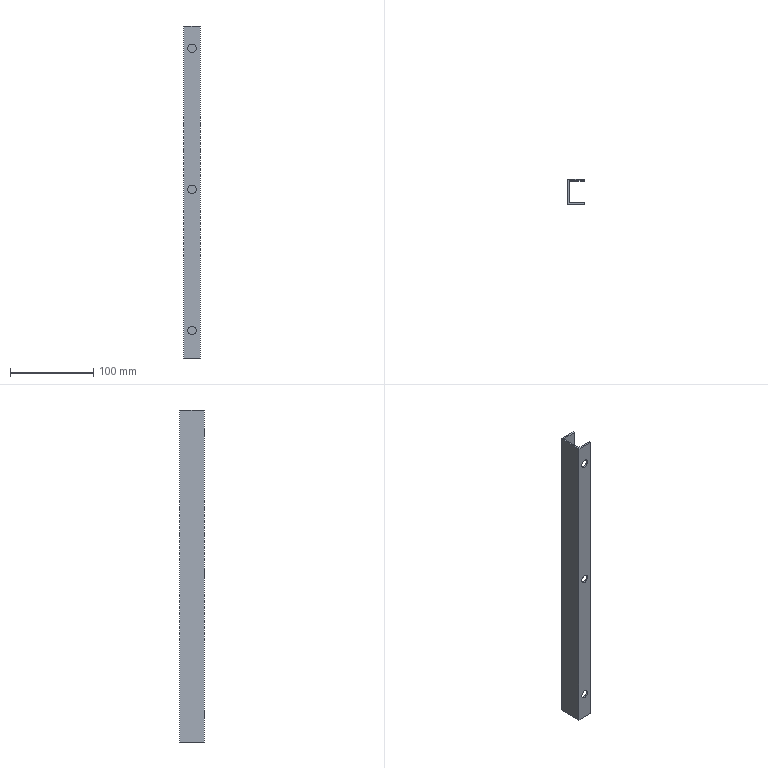Component | SolidWorks | Mirror Part3^Assembly2-4 | 1 solid | 16 faces | box 20 x 30 x 400 mm | volume 52329 mm3 | plane 10 | cylinder 6 | commonest cylinder face diameters 10 x6
STEP:
#1=CARTESIAN_POINT('',(-5.787,0.07874,-30.249));
#2=VERTEX_POINT('',#1);
#3=CARTESIAN_POINT('',(-5.394,0.07874,-30.249));
#4=VERTEX_POINT('',#3);
#5=CARTESIAN_POINT('',(-5.591,0.07874,-30.249));
#6=DIRECTION('',(0.,1.,0.));
#7=DIRECTION('',(-1.,0.,0.));
#8=AXIS2_PLACEMENT_3D('',#5,#6,#7);
#9=CIRCLE('',#8,0.1969);
#10=EDGE_CURVE('',#2,#4,#9,.T.);
#11=ORIENTED_EDGE('',*,*,#10,.T.);
#12=CARTESIAN_POINT('',(-5.394,0.,-30.249));
#13=VERTEX_POINT('',#12);
#14=CARTESIAN_POINT('',(-5.394,0.1969,-30.249));
#15=DIRECTION('',(-0.,-1.,0.));
#16=VECTOR('',#15,39.37);
#17=LINE('',#14,#16);
#18=EDGE_CURVE('',#4,#13,#17,.T.);
#19=ORIENTED_EDGE('',*,*,#18,.T.);
#20=CARTESIAN_POINT('',(-5.787,0.,-30.249));
#21=VERTEX_POINT('',#20);
#22=CARTESIAN_POINT('',(-5.591,0.,-30.249));
#23=DIRECTION('',(0.,1.,0.));
#24=DIRECTION('',(-1.,0.,0.));
#25=AXIS2_PLACEMENT_3D('',#22,#23,#24);
#26=CIRCLE('',#25,0.1969);
#27=EDGE_CURVE('',#21,#13,#26,.T.);
#28=ORIENTED_EDGE('',*,*,#27,.F.);
#29=CARTESIAN_POINT('',(-5.787,0.1969,-30.249));
#30=DIRECTION('',(-0.,-1.,0.));
#31=VECTOR('',#30,39.37);
#32=LINE('',#29,#31);
#33=EDGE_CURVE('',#2,#21,#32,.T.);
#34=ORIENTED_EDGE('',*,*,#33,.F.);
#35=EDGE_LOOP('',(#11,#19,#28,#34));
#36=FACE_OUTER_BOUND('',#35,.T.);
#37=CARTESIAN_POINT('',(-5.591,0.1969,-30.249));
#38=DIRECTION('',(-0.,-1.,0.));
#39=DIRECTION('',(-1.,0.,0.));
#40=AXIS2_PLACEMENT_3D('',#37,#38,#39);
#41=CYLINDRICAL_SURFACE('',#40,0.1969);
#42=ADVANCED_FACE('',(#36),#41,.F.);
#43=CARTESIAN_POINT('',(-5.787,0.07874,-23.556));
#44=VERTEX_POINT('',#43);
#45=CARTESIAN_POINT('',(-5.394,0.07874,-23.556));
#46=VERTEX_POINT('',#45);
#47=CARTESIAN_POINT('',(-5.591,0.07874,-23.556));
#48=DIRECTION('',(0.,1.,0.));
#49=DIRECTION('',(-1.,0.,0.));
#50=AXIS2_PLACEMENT_3D('',#47,#48,#49);
#51=CIRCLE('',#50,0.1969);
#52=EDGE_CURVE('',#44,#46,#51,.T.);
#53=ORIENTED_EDGE('',*,*,#52,.T.);
#54=CARTESIAN_POINT('',(-5.394,0.,-23.556));
#55=VERTEX_POINT('',#54);
#56=CARTESIAN_POINT('',(-5.394,0.1969,-23.556));
#57=DIRECTION('',(-0.,-1.,0.));
#58=VECTOR('',#57,39.37);
#59=LINE('',#56,#58);
#60=EDGE_CURVE('',#46,#55,#59,.T.);
#61=ORIENTED_EDGE('',*,*,#60,.T.);
#62=CARTESIAN_POINT('',(-5.787,0.,-23.556));
#63=VERTEX_POINT('',#62);
#64=CARTESIAN_POINT('',(-5.591,0.,-23.556));
#65=DIRECTION('',(0.,1.,0.));
#66=DIRECTION('',(-1.,0.,0.));
#67=AXIS2_PLACEMENT_3D('',#64,#65,#66);
#68=CIRCLE('',#67,0.1969);
#69=EDGE_CURVE('',#63,#55,#68,.T.);
#70=ORIENTED_EDGE('',*,*,#69,.F.);
#71=CARTESIAN_POINT('',(-5.787,0.1969,-23.556));
#72=DIRECTION('',(-0.,-1.,0.));
#73=VECTOR('',#72,39.37);
#74=LINE('',#71,#73);
#75=EDGE_CURVE('',#44,#63,#74,.T.);
#76=ORIENTED_EDGE('',*,*,#75,.F.);
#77=EDGE_LOOP('',(#53,#61,#70,#76));
#78=FACE_OUTER_BOUND('',#77,.T.);
#79=CARTESIAN_POINT('',(-5.591,0.1969,-23.556));
#80=DIRECTION('',(-0.,-1.,0.));
#81=DIRECTION('',(-1.,0.,0.));
#82=AXIS2_PLACEMENT_3D('',#79,#80,#81);
#83=CYLINDRICAL_SURFACE('',#82,0.1969);
#84=ADVANCED_FACE('',(#78),#83,.F.);
#85=CARTESIAN_POINT('',(-5.787,0.07874,-16.863));
#86=VERTEX_POINT('',#85);
#87=CARTESIAN_POINT('',(-5.394,0.07874,-16.863));
#88=VERTEX_POINT('',#87);
#89=CARTESIAN_POINT('',(-5.591,0.07874,-16.863));
#90=DIRECTION('',(0.,1.,0.));
#91=DIRECTION('',(-1.,0.,0.));
#92=AXIS2_PLACEMENT_3D('',#89,#90,#91);
#93=CIRCLE('',#92,0.1969);
#94=EDGE_CURVE('',#86,#88,#93,.T.);
#95=ORIENTED_EDGE('',*,*,#94,.T.);
#96=CARTESIAN_POINT('',(-5.394,0.,-16.863));
#97=VERTEX_POINT('',#96);
#98=CARTESIAN_POINT('',(-5.394,0.1969,-16.863));
#99=DIRECTION('',(-0.,-1.,0.));
#100=VECTOR('',#99,39.37);
#101=LINE('',#98,#100);
#102=EDGE_CURVE('',#88,#97,#101,.T.);
#103=ORIENTED_EDGE('',*,*,#102,.T.);
#104=CARTESIAN_POINT('',(-5.787,0.,-16.863));
#105=VERTEX_POINT('',#104);
#106=CARTESIAN_POINT('',(-5.591,0.,-16.863));
#107=DIRECTION('',(0.,1.,0.));
#108=DIRECTION('',(-1.,0.,0.));
#109=AXIS2_PLACEMENT_3D('',#106,#107,#108);
#110=CIRCLE('',#109,0.1969);
#111=EDGE_CURVE('',#105,#97,#110,.T.);
#112=ORIENTED_EDGE('',*,*,#111,.F.);
#113=CARTESIAN_POINT('',(-5.787,0.1969,-16.863));
#114=DIRECTION('',(-0.,-1.,0.));
#115=VECTOR('',#114,39.37);
#116=LINE('',#113,#115);
#117=EDGE_CURVE('',#86,#105,#116,.T.);
#118=ORIENTED_EDGE('',*,*,#117,.F.);
#119=EDGE_LOOP('',(#95,#103,#112,#118));
#120=FACE_OUTER_BOUND('',#119,.T.);
#121=CARTESIAN_POINT('',(-5.591,0.1969,-16.863));
#122=DIRECTION('',(-0.,-1.,0.));
#123=DIRECTION('',(-1.,0.,0.));
#124=AXIS2_PLACEMENT_3D('',#121,#122,#123);
#125=CYLINDRICAL_SURFACE('',#124,0.1969);
#126=ADVANCED_FACE('',(#120),#125,.F.);
#127=ORIENTED_EDGE('',*,*,#10,.F.);
#128=CARTESIAN_POINT('',(-5.591,0.07874,-30.249));
#129=DIRECTION('',(0.,1.,0.));
#130=DIRECTION('',(-1.,0.,0.));
#131=AXIS2_PLACEMENT_3D('',#128,#129,#130);
#132=CIRCLE('',#131,0.1969);
#133=EDGE_CURVE('',#4,#2,#132,.T.);
#134=ORIENTED_EDGE('',*,*,#133,.F.);
#135=EDGE_LOOP('',(#127,#134));
#136=FACE_BOUND('',#135,.T.);
#137=ORIENTED_EDGE('',*,*,#52,.F.);
#138=CARTESIAN_POINT('',(-5.591,0.07874,-23.556));
#139=DIRECTION('',(0.,1.,0.));
#140=DIRECTION('',(-1.,0.,0.));
#141=AXIS2_PLACEMENT_3D('',#138,#139,#140);
#142=CIRCLE('',#141,0.1969);
#143=EDGE_CURVE('',#46,#44,#142,.T.);
#144=ORIENTED_EDGE('',*,*,#143,.F.);
#145=EDGE_LOOP('',(#137,#144));
#146=FACE_BOUND('',#145,.T.);
#147=ORIENTED_EDGE('',*,*,#94,.F.);
#148=CARTESIAN_POINT('',(-5.591,0.07874,-16.863));
#149=DIRECTION('',(0.,1.,0.));
#150=DIRECTION('',(-1.,0.,0.));
#151=AXIS2_PLACEMENT_3D('',#148,#149,#150);
#152=CIRCLE('',#151,0.1969);
#153=EDGE_CURVE('',#88,#86,#152,.T.);
#154=ORIENTED_EDGE('',*,*,#153,.F.);
#155=EDGE_LOOP('',(#147,#154));
#156=FACE_BOUND('',#155,.T.);
#157=CARTESIAN_POINT('',(-5.906,0.07874,-31.557));
#158=VERTEX_POINT('',#157);
#159=CARTESIAN_POINT('',(-5.197,0.07874,-31.557));
#160=VERTEX_POINT('',#159);
#161=CARTESIAN_POINT('',(-5.984,0.07874,-31.557));
#162=DIRECTION('',(1.,-0.,0.));
#163=VECTOR('',#162,39.37);
#164=LINE('',#161,#163);
#165=EDGE_CURVE('',#158,#160,#164,.T.);
#166=ORIENTED_EDGE('',*,*,#165,.F.);
#167=CARTESIAN_POINT('',(-5.906,0.07874,-15.809));
#168=VERTEX_POINT('',#167);
#169=CARTESIAN_POINT('',(-5.906,0.07874,-15.809));
#170=DIRECTION('',(0.,0.,-1.));
#171=VECTOR('',#170,39.37);
#172=LINE('',#169,#171);
#173=EDGE_CURVE('',#168,#158,#172,.T.);
#174=ORIENTED_EDGE('',*,*,#173,.F.);
#175=CARTESIAN_POINT('',(-5.197,0.07874,-15.809));
#176=VERTEX_POINT('',#175);
#177=CARTESIAN_POINT('',(-5.984,0.07874,-15.809));
#178=DIRECTION('',(1.,-0.,0.));
#179=VECTOR('',#178,39.37);
#180=LINE('',#177,#179);
#181=EDGE_CURVE('',#168,#176,#180,.T.);
#182=ORIENTED_EDGE('',*,*,#181,.T.);
#183=CARTESIAN_POINT('',(-5.197,0.07874,-15.809));
#184=DIRECTION('',(0.,0.,-1.));
#185=VECTOR('',#184,39.37);
#186=LINE('',#183,#185);
#187=EDGE_CURVE('',#176,#160,#186,.T.);
#188=ORIENTED_EDGE('',*,*,#187,.T.);
#189=EDGE_LOOP('',(#166,#174,#182,#188));
#190=FACE_OUTER_BOUND('',#189,.T.);
#191=CARTESIAN_POINT('',(-5.984,0.07874,-15.809));
#192=DIRECTION('',(-0.,-1.,0.));
#193=DIRECTION('',(-1.,0.,0.));
#194=AXIS2_PLACEMENT_3D('',#191,#192,#193);
#195=PLANE('',#194);
#196=ADVANCED_FACE('',(#136,#146,#156,#190),#195,.F.);
#197=CARTESIAN_POINT('',(-5.197,0.,-31.557));
#198=VERTEX_POINT('',#197);
#199=CARTESIAN_POINT('',(-5.197,0.,-31.557));
#200=DIRECTION('',(0.,1.,0.));
#201=VECTOR('',#200,39.37);
#202=LINE('',#199,#201);
#203=EDGE_CURVE('',#198,#160,#202,.T.);
#204=ORIENTED_EDGE('',*,*,#203,.T.);
#205=ORIENTED_EDGE('',*,*,#187,.F.);
#206=CARTESIAN_POINT('',(-5.197,0.,-15.809));
#207=VERTEX_POINT('',#206);
#208=CARTESIAN_POINT('',(-5.197,0.,-15.809));
#209=DIRECTION('',(0.,1.,0.));
#210=VECTOR('',#209,39.37);
#211=LINE('',#208,#210);
#212=EDGE_CURVE('',#207,#176,#211,.T.);
#213=ORIENTED_EDGE('',*,*,#212,.F.);
#214=CARTESIAN_POINT('',(-5.197,0.,-15.809));
#215=DIRECTION('',(0.,0.,-1.));
#216=VECTOR('',#215,39.37);
#217=LINE('',#214,#216);
#218=EDGE_CURVE('',#207,#198,#217,.T.);
#219=ORIENTED_EDGE('',*,*,#218,.T.);
#220=EDGE_LOOP('',(#204,#205,#213,#219));
#221=FACE_OUTER_BOUND('',#220,.T.);
#222=CARTESIAN_POINT('',(-5.197,0.,-15.809));
#223=DIRECTION('',(1.,0.,0.));
#224=DIRECTION('',(0.,0.,1.));
#225=AXIS2_PLACEMENT_3D('',#222,#223,#224);
#226=PLANE('',#225);
#227=ADVANCED_FACE('',(#221),#226,.T.);
#228=ORIENTED_EDGE('',*,*,#27,.T.);
#229=CARTESIAN_POINT('',(-5.591,0.,-30.249));
#230=DIRECTION('',(0.,1.,0.));
#231=DIRECTION('',(-1.,0.,0.));
#232=AXIS2_PLACEMENT_3D('',#229,#230,#231);
#233=CIRCLE('',#232,0.1969);
#234=EDGE_CURVE('',#13,#21,#233,.T.);
#235=ORIENTED_EDGE('',*,*,#234,.T.);
#236=EDGE_LOOP('',(#228,#235));
#237=FACE_BOUND('',#236,.T.);
#238=ORIENTED_EDGE('',*,*,#69,.T.);
#239=CARTESIAN_POINT('',(-5.591,0.,-23.556));
#240=DIRECTION('',(0.,1.,0.));
#241=DIRECTION('',(-1.,0.,0.));
#242=AXIS2_PLACEMENT_3D('',#239,#240,#241);
#243=CIRCLE('',#242,0.1969);
#244=EDGE_CURVE('',#55,#63,#243,.T.);
#245=ORIENTED_EDGE('',*,*,#244,.T.);
#246=EDGE_LOOP('',(#238,#245));
#247=FACE_BOUND('',#246,.T.);
#248=ORIENTED_EDGE('',*,*,#111,.T.);
#249=CARTESIAN_POINT('',(-5.591,0.,-16.863));
#250=DIRECTION('',(0.,1.,0.));
#251=DIRECTION('',(-1.,0.,0.));
#252=AXIS2_PLACEMENT_3D('',#249,#250,#251);
#253=CIRCLE('',#252,0.1969);
#254=EDGE_CURVE('',#97,#105,#253,.T.);
#255=ORIENTED_EDGE('',*,*,#254,.T.);
#256=EDGE_LOOP('',(#248,#255));
#257=FACE_BOUND('',#256,.T.);
#258=CARTESIAN_POINT('',(-5.984,0.,-31.557));
#259=VERTEX_POINT('',#258);
#260=CARTESIAN_POINT('',(-5.984,0.,-31.557));
#261=DIRECTION('',(1.,-0.,0.));
#262=VECTOR('',#261,39.37);
#263=LINE('',#260,#262);
#264=EDGE_CURVE('',#259,#198,#263,.T.);
#265=ORIENTED_EDGE('',*,*,#264,.T.);
#266=ORIENTED_EDGE('',*,*,#218,.F.);
#267=CARTESIAN_POINT('',(-5.984,0.,-15.809));
#268=VERTEX_POINT('',#267);
#269=CARTESIAN_POINT('',(-5.984,0.,-15.809));
#270=DIRECTION('',(1.,-0.,0.));
#271=VECTOR('',#270,39.37);
#272=LINE('',#269,#271);
#273=EDGE_CURVE('',#268,#207,#272,.T.);
#274=ORIENTED_EDGE('',*,*,#273,.F.);
#275=CARTESIAN_POINT('',(-5.984,0.,-15.809));
#276=DIRECTION('',(0.,0.,-1.));
#277=VECTOR('',#276,39.37);
#278=LINE('',#275,#277);
#279=EDGE_CURVE('',#268,#259,#278,.T.);
#280=ORIENTED_EDGE('',*,*,#279,.T.);
#281=EDGE_LOOP('',(#265,#266,#274,#280));
#282=FACE_OUTER_BOUND('',#281,.T.);
#283=CARTESIAN_POINT('',(-5.984,0.,-15.809));
#284=DIRECTION('',(-0.,-1.,0.));
#285=DIRECTION('',(-1.,0.,0.));
#286=AXIS2_PLACEMENT_3D('',#283,#284,#285);
#287=PLANE('',#286);
#288=ADVANCED_FACE('',(#237,#247,#257,#282),#287,.T.);
#289=CARTESIAN_POINT('',(-5.984,1.181,-31.557));
#290=VERTEX_POINT('',#289);
#291=CARTESIAN_POINT('',(-5.984,0.,-31.557));
#292=DIRECTION('',(0.,-1.,0.));
#293=VECTOR('',#292,39.37);
#294=LINE('',#291,#293);
#295=EDGE_CURVE('',#290,#259,#294,.T.);
#296=ORIENTED_EDGE('',*,*,#295,.T.);
#297=ORIENTED_EDGE('',*,*,#279,.F.);
#298=CARTESIAN_POINT('',(-5.984,1.181,-15.809));
#299=VERTEX_POINT('',#298);
#300=CARTESIAN_POINT('',(-5.984,0.,-15.809));
#301=DIRECTION('',(0.,-1.,0.));
#302=VECTOR('',#301,39.37);
#303=LINE('',#300,#302);
#304=EDGE_CURVE('',#299,#268,#303,.T.);
#305=ORIENTED_EDGE('',*,*,#304,.F.);
#306=CARTESIAN_POINT('',(-5.984,1.181,-15.809));
#307=DIRECTION('',(0.,0.,-1.));
#308=VECTOR('',#307,39.37);
#309=LINE('',#306,#308);
#310=EDGE_CURVE('',#299,#290,#309,.T.);
#311=ORIENTED_EDGE('',*,*,#310,.T.);
#312=EDGE_LOOP('',(#296,#297,#305,#311));
#313=FACE_OUTER_BOUND('',#312,.T.);
#314=CARTESIAN_POINT('',(-5.984,0.,-15.809));
#315=DIRECTION('',(-1.,0.,0.));
#316=DIRECTION('',(0.,0.,-1.));
#317=AXIS2_PLACEMENT_3D('',#314,#315,#316);
#318=PLANE('',#317);
#319=ADVANCED_FACE('',(#313),#318,.T.);
#320=CARTESIAN_POINT('',(-5.197,1.181,-31.557));
#321=VERTEX_POINT('',#320);
#322=CARTESIAN_POINT('',(-5.984,1.181,-31.557));
#323=DIRECTION('',(-1.,0.,0.));
#324=VECTOR('',#323,39.37);
#325=LINE('',#322,#324);
#326=EDGE_CURVE('',#321,#290,#325,.T.);
#327=ORIENTED_EDGE('',*,*,#326,.T.);
#328=ORIENTED_EDGE('',*,*,#310,.F.);
#329=CARTESIAN_POINT('',(-5.197,1.181,-15.809));
#330=VERTEX_POINT('',#329);
#331=CARTESIAN_POINT('',(-5.984,1.181,-15.809));
#332=DIRECTION('',(-1.,0.,0.));
#333=VECTOR('',#332,39.37);
#334=LINE('',#331,#333);
#335=EDGE_CURVE('',#330,#299,#334,.T.);
#336=ORIENTED_EDGE('',*,*,#335,.F.);
#337=CARTESIAN_POINT('',(-5.197,1.181,-15.809));
#338=DIRECTION('',(0.,0.,-1.));
#339=VECTOR('',#338,39.37);
#340=LINE('',#337,#339);
#341=EDGE_CURVE('',#330,#321,#340,.T.);
#342=ORIENTED_EDGE('',*,*,#341,.T.);
#343=EDGE_LOOP('',(#327,#328,#336,#342));
#344=FACE_OUTER_BOUND('',#343,.T.);
#345=CARTESIAN_POINT('',(-5.984,1.181,-15.809));
#346=DIRECTION('',(0.,1.,0.));
#347=DIRECTION('',(0.,0.,1.));
#348=AXIS2_PLACEMENT_3D('',#345,#346,#347);
#349=PLANE('',#348);
#350=ADVANCED_FACE('',(#344),#349,.T.);
#351=CARTESIAN_POINT('',(-5.197,1.102,-31.557));
#352=VERTEX_POINT('',#351);
#353=CARTESIAN_POINT('',(-5.197,1.102,-31.557));
#354=DIRECTION('',(0.,1.,0.));
#355=VECTOR('',#354,39.37);
#356=LINE('',#353,#355);
#357=EDGE_CURVE('',#352,#321,#356,.T.);
#358=ORIENTED_EDGE('',*,*,#357,.T.);
#359=ORIENTED_EDGE('',*,*,#341,.F.);
#360=CARTESIAN_POINT('',(-5.197,1.102,-15.809));
#361=VERTEX_POINT('',#360);
#362=CARTESIAN_POINT('',(-5.197,1.102,-15.809));
#363=DIRECTION('',(0.,1.,0.));
#364=VECTOR('',#363,39.37);
#365=LINE('',#362,#364);
#366=EDGE_CURVE('',#361,#330,#365,.T.);
#367=ORIENTED_EDGE('',*,*,#366,.F.);
#368=CARTESIAN_POINT('',(-5.197,1.102,-15.809));
#369=DIRECTION('',(0.,0.,-1.));
#370=VECTOR('',#369,39.37);
#371=LINE('',#368,#370);
#372=EDGE_CURVE('',#361,#352,#371,.T.);
#373=ORIENTED_EDGE('',*,*,#372,.T.);
#374=EDGE_LOOP('',(#358,#359,#367,#373));
#375=FACE_OUTER_BOUND('',#374,.T.);
#376=CARTESIAN_POINT('',(-5.197,1.102,-15.809));
#377=DIRECTION('',(1.,0.,0.));
#378=DIRECTION('',(0.,0.,1.));
#379=AXIS2_PLACEMENT_3D('',#376,#377,#378);
#380=PLANE('',#379);
#381=ADVANCED_FACE('',(#375),#380,.T.);
#382=CARTESIAN_POINT('',(-5.906,1.102,-31.557));
#383=VERTEX_POINT('',#382);
#384=CARTESIAN_POINT('',(-5.984,1.102,-31.557));
#385=DIRECTION('',(-1.,0.,0.));
#386=VECTOR('',#385,39.37);
#387=LINE('',#384,#386);
#388=EDGE_CURVE('',#352,#383,#387,.T.);
#389=ORIENTED_EDGE('',*,*,#388,.F.);
#390=ORIENTED_EDGE('',*,*,#372,.F.);
#391=CARTESIAN_POINT('',(-5.906,1.102,-15.809));
#392=VERTEX_POINT('',#391);
#393=CARTESIAN_POINT('',(-5.984,1.102,-15.809));
#394=DIRECTION('',(-1.,0.,0.));
#395=VECTOR('',#394,39.37);
#396=LINE('',#393,#395);
#397=EDGE_CURVE('',#361,#392,#396,.T.);
#398=ORIENTED_EDGE('',*,*,#397,.T.);
#399=CARTESIAN_POINT('',(-5.906,1.102,-15.809));
#400=DIRECTION('',(0.,0.,-1.));
#401=VECTOR('',#400,39.37);
#402=LINE('',#399,#401);
#403=EDGE_CURVE('',#392,#383,#402,.T.);
#404=ORIENTED_EDGE('',*,*,#403,.T.);
#405=EDGE_LOOP('',(#389,#390,#398,#404));
#406=FACE_OUTER_BOUND('',#405,.T.);
#407=CARTESIAN_POINT('',(-5.984,1.102,-15.809));
#408=DIRECTION('',(0.,1.,0.));
#409=DIRECTION('',(0.,0.,1.));
#410=AXIS2_PLACEMENT_3D('',#407,#408,#409);
#411=PLANE('',#410);
#412=ADVANCED_FACE('',(#406),#411,.F.);
#413=CARTESIAN_POINT('',(-5.906,0.,-31.557));
#414=DIRECTION('',(0.,-1.,0.));
#415=VECTOR('',#414,39.37);
#416=LINE('',#413,#415);
#417=EDGE_CURVE('',#383,#158,#416,.T.);
#418=ORIENTED_EDGE('',*,*,#417,.F.);
#419=ORIENTED_EDGE('',*,*,#403,.F.);
#420=CARTESIAN_POINT('',(-5.906,0.,-15.809));
#421=DIRECTION('',(0.,-1.,0.));
#422=VECTOR('',#421,39.37);
#423=LINE('',#420,#422);
#424=EDGE_CURVE('',#392,#168,#423,.T.);
#425=ORIENTED_EDGE('',*,*,#424,.T.);
#426=ORIENTED_EDGE('',*,*,#173,.T.);
#427=EDGE_LOOP('',(#418,#419,#425,#426));
#428=FACE_OUTER_BOUND('',#427,.T.);
#429=CARTESIAN_POINT('',(-5.906,0.,-15.809));
#430=DIRECTION('',(-1.,0.,0.));
#431=DIRECTION('',(0.,0.,-1.));
#432=AXIS2_PLACEMENT_3D('',#429,#430,#431);
#433=PLANE('',#432);
#434=ADVANCED_FACE('',(#428),#433,.F.);
#435=ORIENTED_EDGE('',*,*,#181,.F.);
#436=ORIENTED_EDGE('',*,*,#424,.F.);
#437=ORIENTED_EDGE('',*,*,#397,.F.);
#438=ORIENTED_EDGE('',*,*,#366,.T.);
#439=ORIENTED_EDGE('',*,*,#335,.T.);
#440=ORIENTED_EDGE('',*,*,#304,.T.);
#441=ORIENTED_EDGE('',*,*,#273,.T.);
#442=ORIENTED_EDGE('',*,*,#212,.T.);
#443=EDGE_LOOP('',(#435,#436,#437,#438,#439,#440,#441,#442));
#444=FACE_OUTER_BOUND('',#443,.T.);
#445=CARTESIAN_POINT('',(-5.984,0.5561,-15.809));
#446=DIRECTION('',(0.,0.,-1.));
#447=DIRECTION('',(1.,0.,0.));
#448=AXIS2_PLACEMENT_3D('',#445,#446,#447);
#449=PLANE('',#448);
#450=ADVANCED_FACE('',(#444),#449,.F.);
#451=ORIENTED_EDGE('',*,*,#165,.T.);
#452=ORIENTED_EDGE('',*,*,#203,.F.);
#453=ORIENTED_EDGE('',*,*,#264,.F.);
#454=ORIENTED_EDGE('',*,*,#295,.F.);
#455=ORIENTED_EDGE('',*,*,#326,.F.);
#456=ORIENTED_EDGE('',*,*,#357,.F.);
#457=ORIENTED_EDGE('',*,*,#388,.T.);
#458=ORIENTED_EDGE('',*,*,#417,.T.);
#459=EDGE_LOOP('',(#451,#452,#453,#454,#455,#456,#457,#458));
#460=FACE_OUTER_BOUND('',#459,.T.);
#461=CARTESIAN_POINT('',(-5.984,0.5561,-31.557));
#462=DIRECTION('',(0.,0.,-1.));
#463=DIRECTION('',(1.,0.,0.));
#464=AXIS2_PLACEMENT_3D('',#461,#462,#463);
#465=PLANE('',#464);
#466=ADVANCED_FACE('',(#460),#465,.T.);
#467=ORIENTED_EDGE('',*,*,#102,.F.);
#468=ORIENTED_EDGE('',*,*,#153,.T.);
#469=ORIENTED_EDGE('',*,*,#117,.T.);
#470=ORIENTED_EDGE('',*,*,#254,.F.);
#471=EDGE_LOOP('',(#467,#468,#469,#470));
#472=FACE_OUTER_BOUND('',#471,.T.);
#473=CARTESIAN_POINT('',(-5.591,0.1969,-16.863));
#474=DIRECTION('',(-0.,-1.,0.));
#475=DIRECTION('',(-1.,0.,0.));
#476=AXIS2_PLACEMENT_3D('',#473,#474,#475);
#477=CYLINDRICAL_SURFACE('',#476,0.1969);
#478=ADVANCED_FACE('',(#472),#477,.F.);
#479=ORIENTED_EDGE('',*,*,#60,.F.);
#480=ORIENTED_EDGE('',*,*,#143,.T.);
#481=ORIENTED_EDGE('',*,*,#75,.T.);
#482=ORIENTED_EDGE('',*,*,#244,.F.);
#483=EDGE_LOOP('',(#479,#480,#481,#482));
#484=FACE_OUTER_BOUND('',#483,.T.);
#485=CARTESIAN_POINT('',(-5.591,0.1969,-23.556));
#486=DIRECTION('',(-0.,-1.,0.));
#487=DIRECTION('',(-1.,0.,0.));
#488=AXIS2_PLACEMENT_3D('',#485,#486,#487);
#489=CYLINDRICAL_SURFACE('',#488,0.1969);
#490=ADVANCED_FACE('',(#484),#489,.F.);
#491=ORIENTED_EDGE('',*,*,#18,.F.);
#492=ORIENTED_EDGE('',*,*,#133,.T.);
#493=ORIENTED_EDGE('',*,*,#33,.T.);
#494=ORIENTED_EDGE('',*,*,#234,.F.);
#495=EDGE_LOOP('',(#491,#492,#493,#494));
#496=FACE_OUTER_BOUND('',#495,.T.);
#497=CARTESIAN_POINT('',(-5.591,0.1969,-30.249));
#498=DIRECTION('',(-0.,-1.,0.));
#499=DIRECTION('',(-1.,0.,0.));
#500=AXIS2_PLACEMENT_3D('',#497,#498,#499);
#501=CYLINDRICAL_SURFACE('',#500,0.1969);
#502=ADVANCED_FACE('',(#496),#501,.F.);
#503=CLOSED_SHELL('',(#42,#84,#126,#196,#227,#288,#319,#350,#381,#412,#434,#450,#466,#478,#490,#502));
#504=MANIFOLD_SOLID_BREP('',#503);
#505=CARTESIAN_POINT('',(0.,0.,0.));
#506=DIRECTION('',(0.,0.,1.));
#507=DIRECTION('',(1.,0.,0.));
#508=AXIS2_PLACEMENT_3D('',#505,#506,#507);
#509=(LENGTH_UNIT()NAMED_UNIT(*)SI_UNIT($,.METRE.));
#510=LENGTH_MEASURE_WITH_UNIT(LENGTH_MEASURE(0.0254),#509);
#511=DIMENSIONAL_EXPONENTS(1.,0.,0.,0.,0.,0.,0.);
#512=(CONVERSION_BASED_UNIT('',#510)LENGTH_UNIT()NAMED_UNIT(#511));
#513=UNCERTAINTY_MEASURE_WITH_UNIT(LENGTH_MEASURE(0.00001),#512,'','');
#514=(NAMED_UNIT(*)PLANE_ANGLE_UNIT()SI_UNIT($,.RADIAN.));
#515=(NAMED_UNIT(*)SI_UNIT($,.STERADIAN.)SOLID_ANGLE_UNIT());
#516=(GEOMETRIC_REPRESENTATION_CONTEXT(3)GLOBAL_UNCERTAINTY_ASSIGNED_CONTEXT((#513))GLOBAL_UNIT_ASSIGNED_CONTEXT((#512,#514,#515))REPRESENTATION_CONTEXT('',''));
#517=ADVANCED_BREP_SHAPE_REPRESENTATION('',(#504,#508),#516);
#518=COLOUR_RGB('',0.7922,0.8196,0.9333);
#519=FILL_AREA_STYLE_COLOUR('',#518);
#520=FILL_AREA_STYLE('',(#519));
#521=SURFACE_STYLE_FILL_AREA(#520);
#522=SURFACE_SIDE_STYLE('',(#521));
#523=SURFACE_STYLE_USAGE(.BOTH.,#522);
#524=PRESENTATION_STYLE_ASSIGNMENT((#523));
#525=STYLED_ITEM('',(#524),#504);
#526=(LENGTH_UNIT()NAMED_UNIT(*)SI_UNIT($,.METRE.));
#527=LENGTH_MEASURE_WITH_UNIT(LENGTH_MEASURE(0.0254),#526);
#528=DIMENSIONAL_EXPONENTS(1.,0.,0.,0.,0.,0.,0.);
#529=(CONVERSION_BASED_UNIT('',#527)LENGTH_UNIT()NAMED_UNIT(#528));
#530=UNCERTAINTY_MEASURE_WITH_UNIT(LENGTH_MEASURE(0.00001),#529,'','');
#531=(NAMED_UNIT(*)PLANE_ANGLE_UNIT()SI_UNIT($,.RADIAN.));
#532=(NAMED_UNIT(*)SI_UNIT($,.STERADIAN.)SOLID_ANGLE_UNIT());
#533=(GEOMETRIC_REPRESENTATION_CONTEXT(3)GLOBAL_UNCERTAINTY_ASSIGNED_CONTEXT((#530))GLOBAL_UNIT_ASSIGNED_CONTEXT((#529,#531,#532))REPRESENTATION_CONTEXT('',''));
#534=MECHANICAL_DESIGN_GEOMETRIC_PRESENTATION_REPRESENTATION('',(#525),#533);
#535=PRESENTATION_LAYER_ASSIGNMENT('','',(#525));